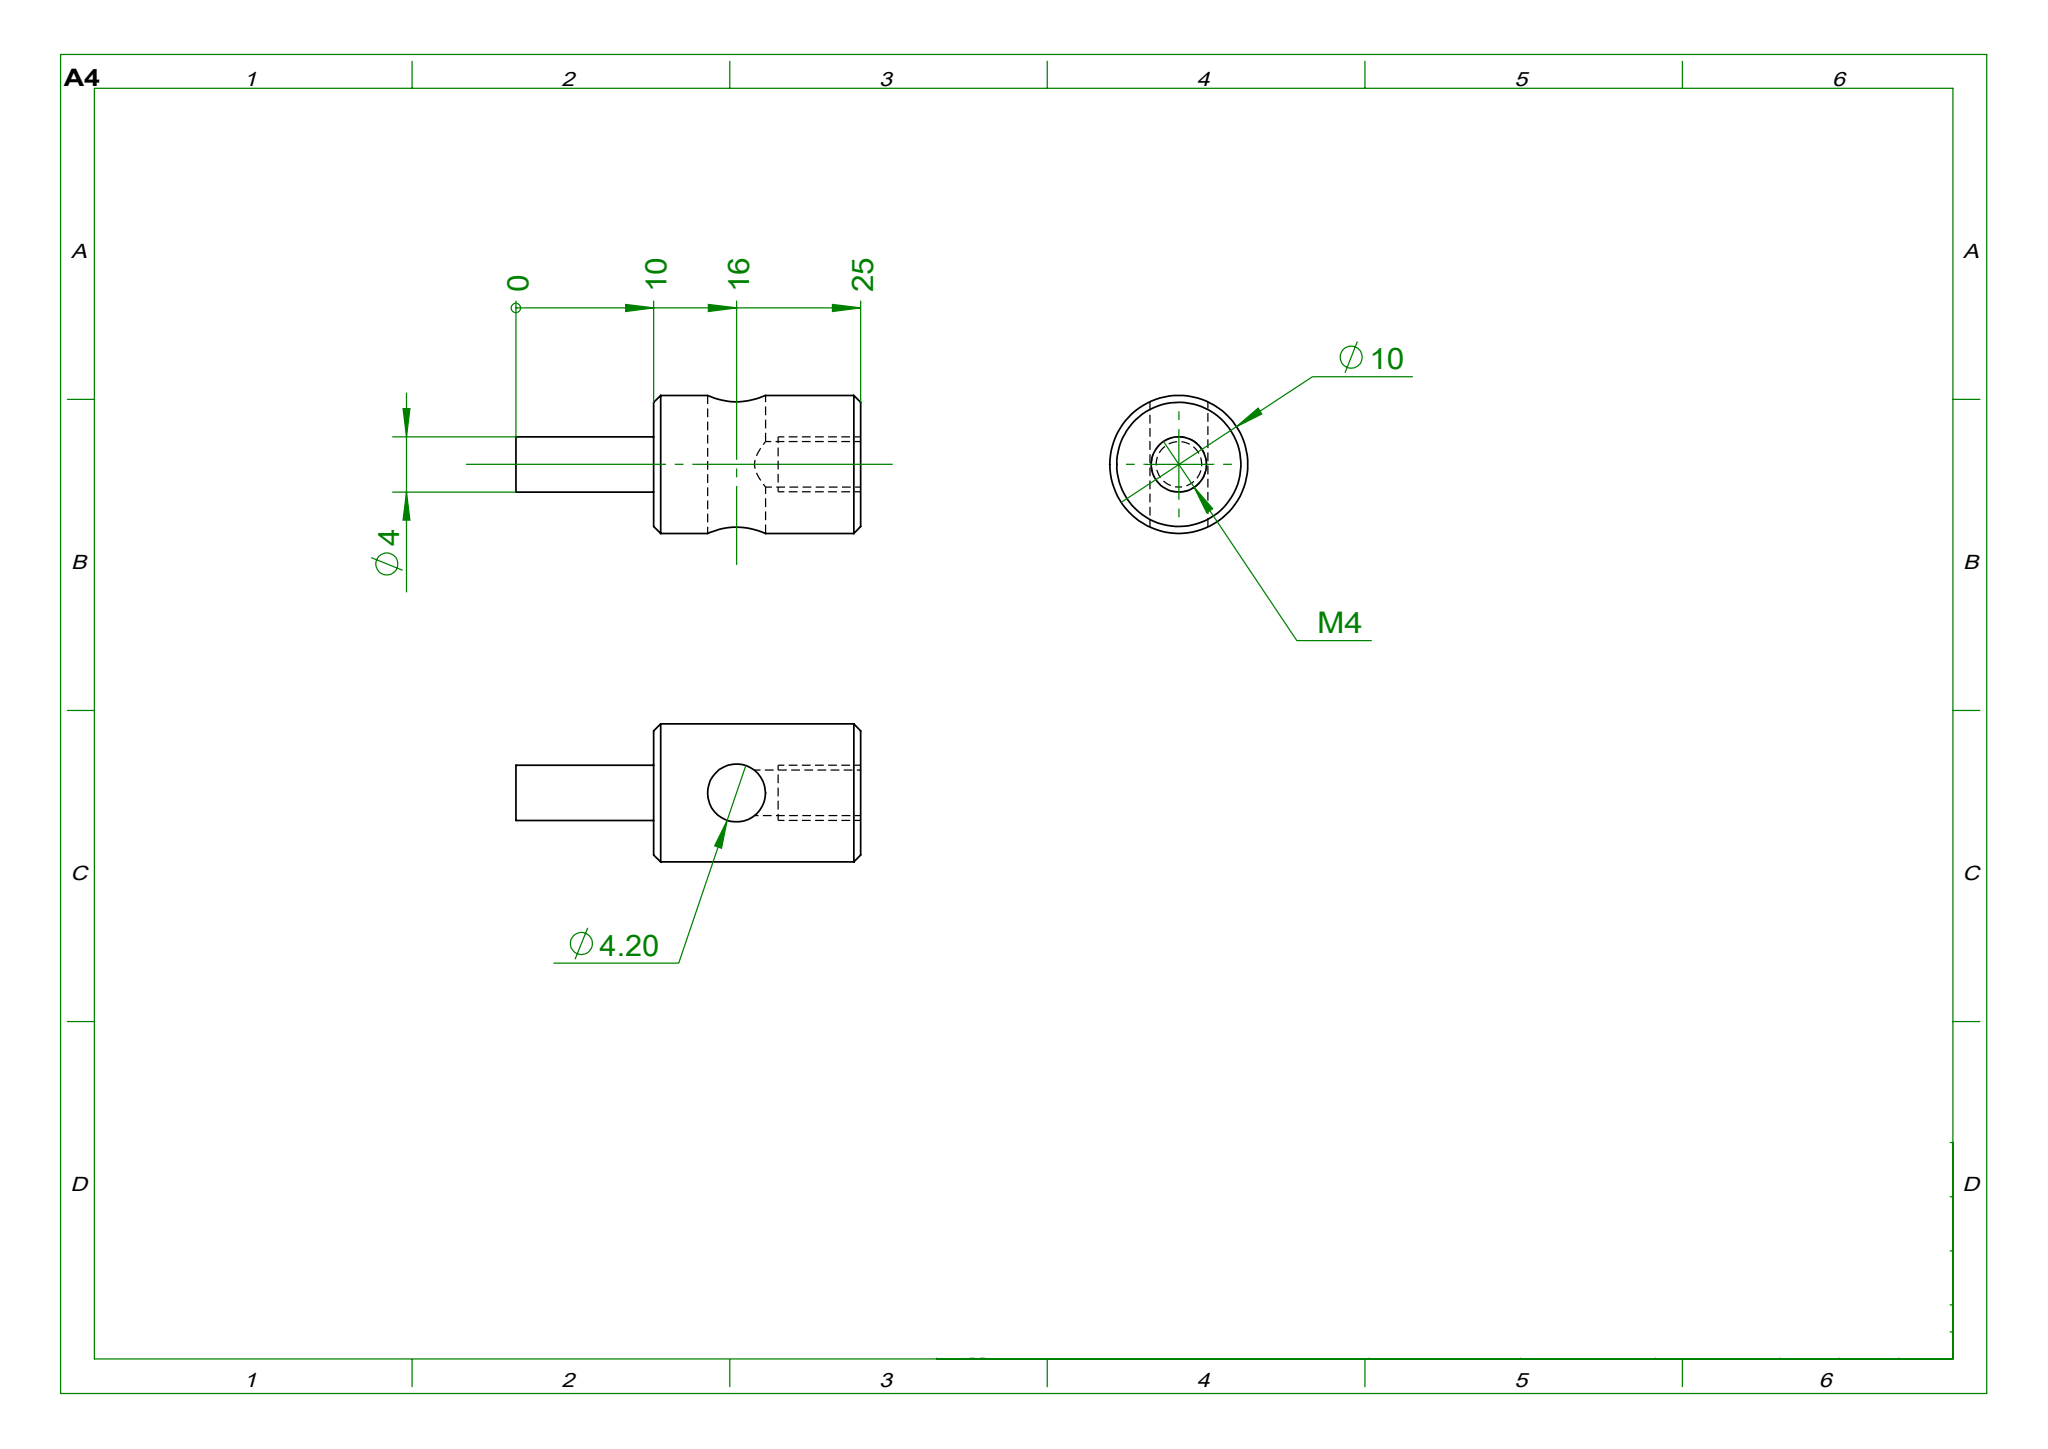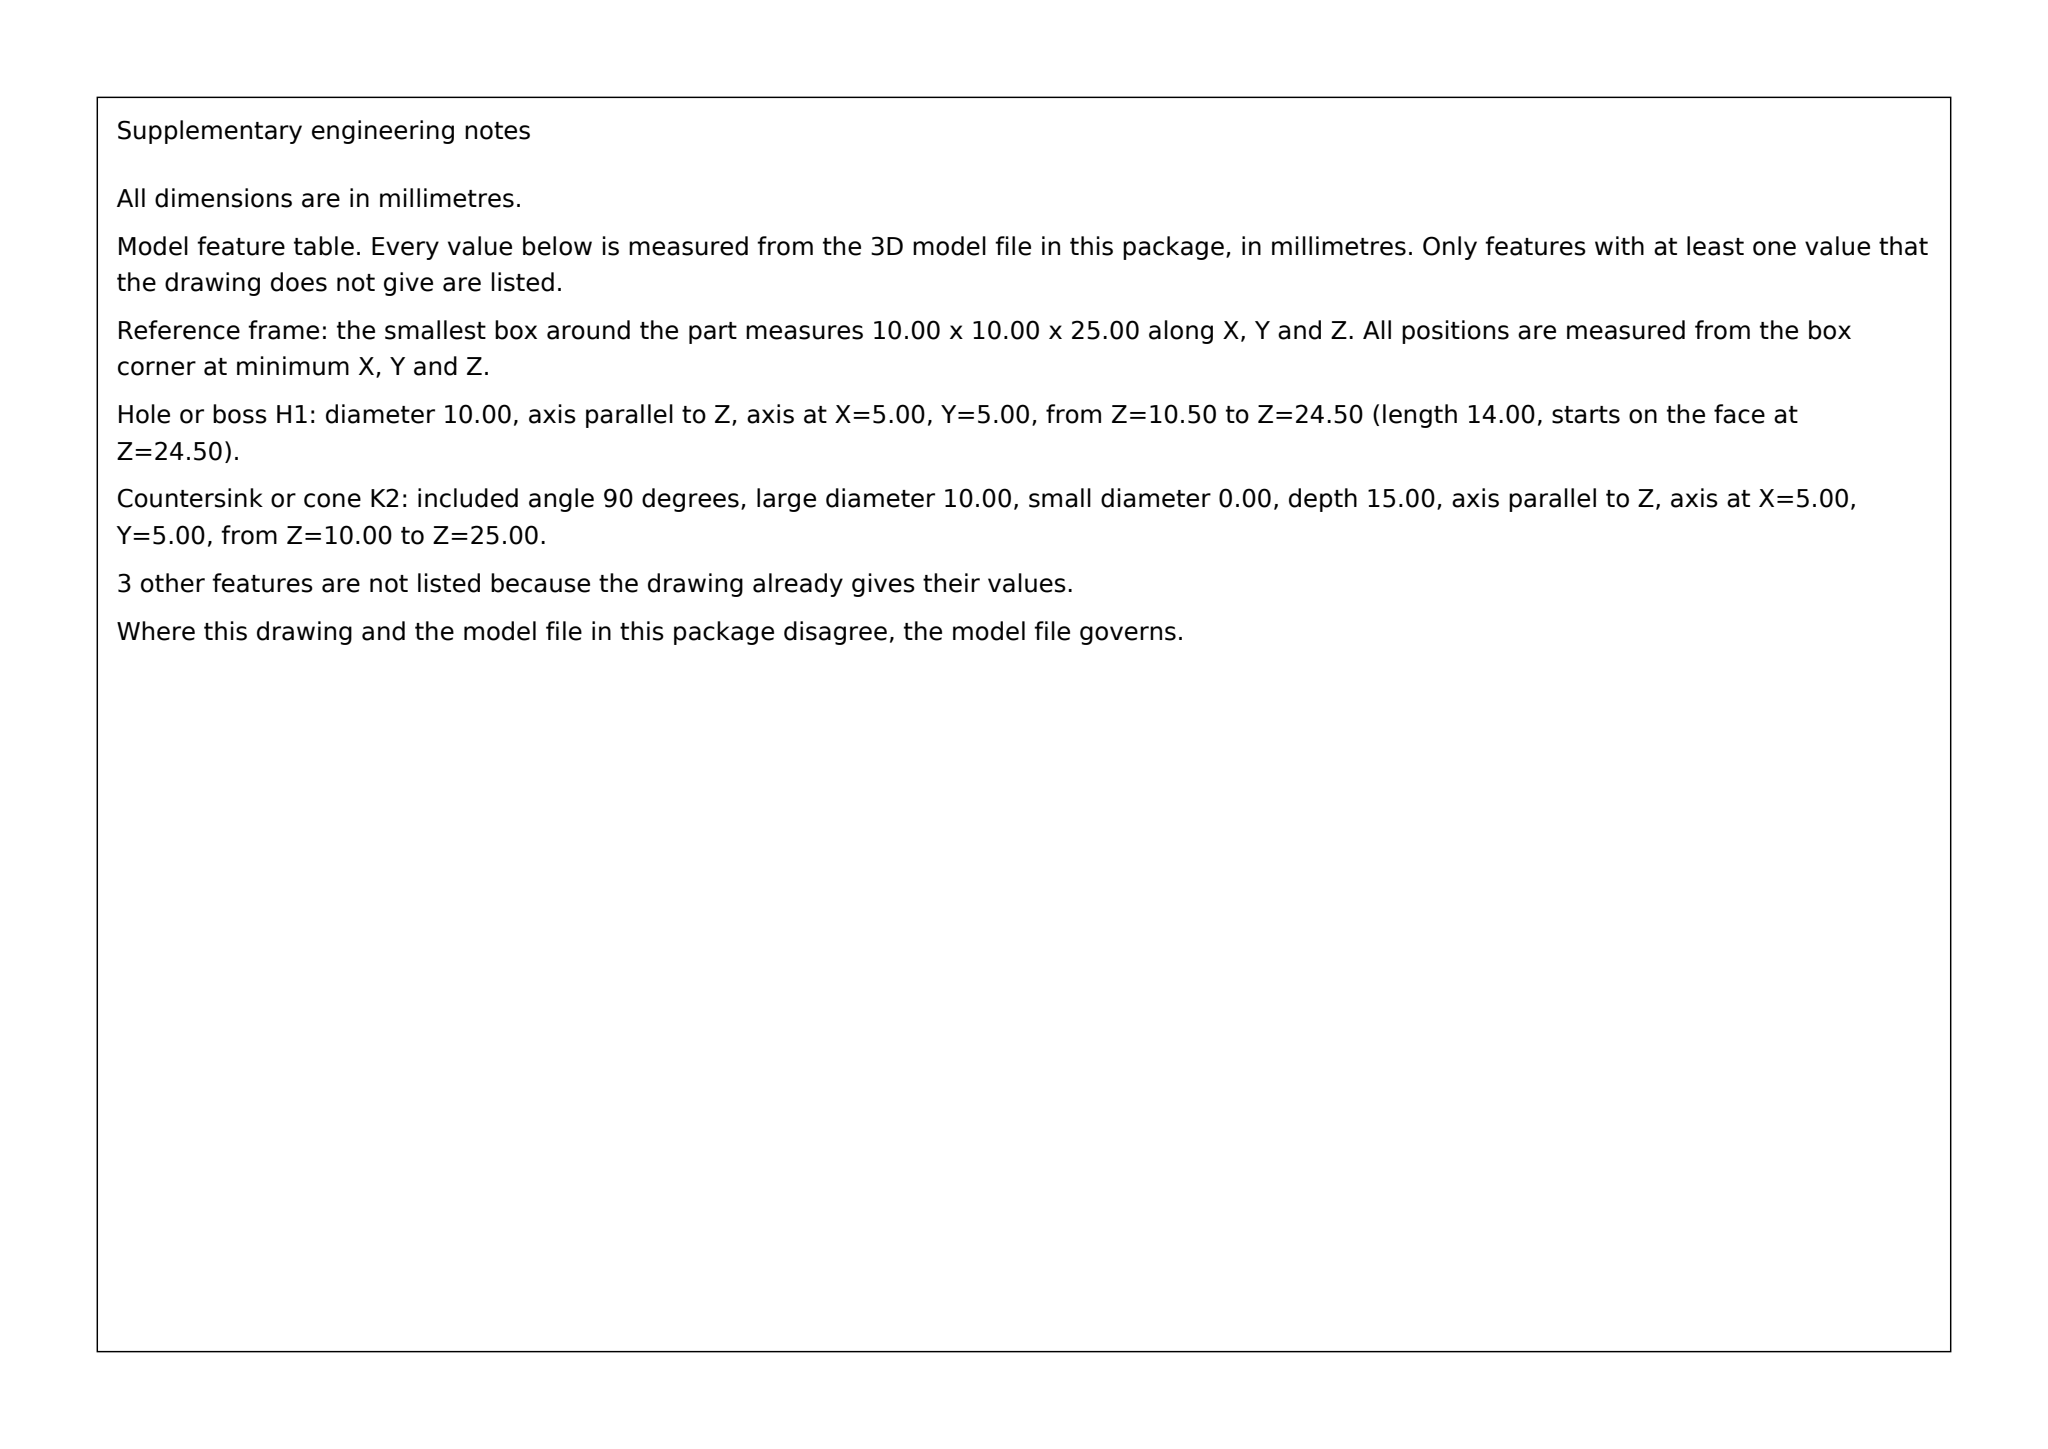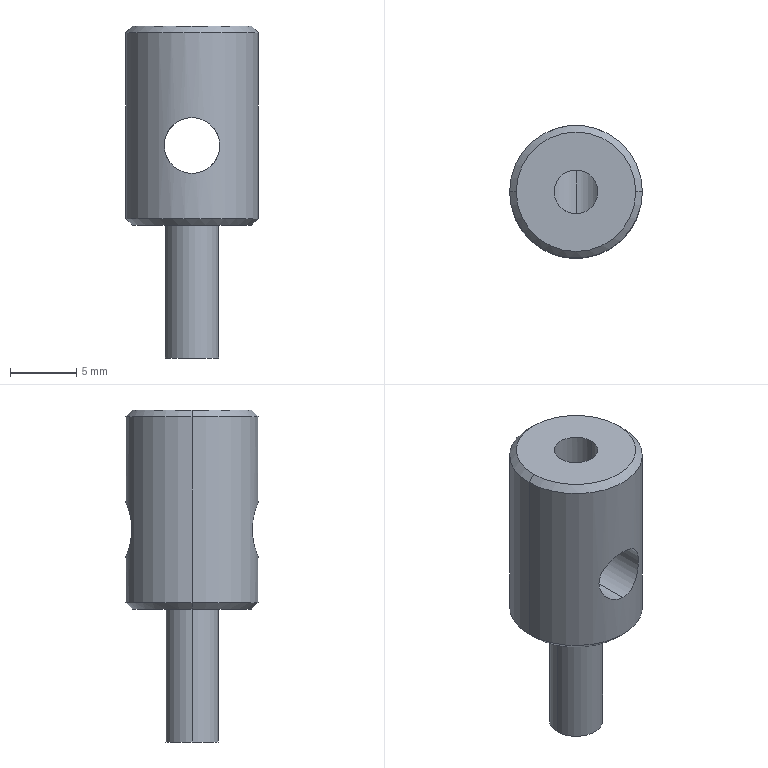Part | SolidWorks | mm | 1 solid | 15 faces | box 10 x 10 x 25 mm | volume 1100 mm3 | cylinder 8 | cone 4 | plane 3 | commonest cylinder face diameters 3.3 x2 4.2 x2 10 x2 4 x2
Drawing notes:
M4 DP 7.7, TAP DRILL Ø3.3 DP 7.7 FROM Ø10 END FACE (25) | from the solid: Ø3.3 z-axis cyl at (5,5), L=7.7 from z=25 face; Ø10 end face plane z=25
Ø10 END: CHAMFER 0.5 X 45° (Ø10 TO Ø9) | from the solid: cones 90° incl, ref Ø10 and Ø9 at Ø10 end; Ø10 cyl L=14 over 15 span
UNSPEC CHAMFERS 0.5 X 45°, BREAK SHARP EDGES | from the solid: only 90° included-angle cones Ø10/Ø9 present; no fillet radii in model
build123d program:
from build123d import *

# Parameters (mm, degrees)
SKETCH1_R             = 2
BOSS_EXTRUDE1_DEPTH   = 10
SKETCH2_R             = 5
BOSS_EXTRUDE2_DEPTH   = 15
SKETCH3_R             = 2.1
CUT_EXTRUDE1_DEPTH    = 6
M4_TAPPED_HOLE1_D     = 3.3
M4_TAPPED_HOLE1_DEPTH = 8
M4_TAPPED_HOLE1_TIP   = 0.9914
CHAMFER1_SIZE         = 0.5


with BuildPart() as part:
    # Sketch1 → Boss-Extrude1 (new body)
    with BuildSketch(Plane.XY):
        Circle(SKETCH1_R)
    extrude(amount=BOSS_EXTRUDE1_DEPTH)

    # Sketch2 → Boss-Extrude2 (add)
    with BuildSketch(Plane.XY.offset(10)):
        Circle(SKETCH2_R)
    extrude(amount=BOSS_EXTRUDE2_DEPTH)

    # Sketch3 → Cut-Extrude1 (cut, symmetric)
    with BuildSketch(Plane(origin=(0, 0, 0), x_dir=(1, 0, 0), z_dir=(0, 1, 0))):
        with Locations(Location((0, -16, 0), (0, 0, 270))):
            Circle(SKETCH3_R)
    extrude(amount=CUT_EXTRUDE1_DEPTH, both=True, mode=Mode.SUBTRACT)

    # M4 Tapped Hole1
    with Locations(Plane.XY.offset(25)):
        with Locations((0, 0)):
            Hole(M4_TAPPED_HOLE1_D / 2, depth=M4_TAPPED_HOLE1_DEPTH)
            with Locations((0, 0, -(M4_TAPPED_HOLE1_DEPTH + M4_TAPPED_HOLE1_TIP / 2))):  # 118° drill point
                Cone(0, M4_TAPPED_HOLE1_D / 2, M4_TAPPED_HOLE1_TIP, mode=Mode.SUBTRACT)

    # Chamfer1
    chamfer1_edges = [part.edges().sort_by_distance(p)[0] for p in [
        (-5, 0, 10),
        (-5, 0, 25),
    ]]
    chamfer(chamfer1_edges, length=CHAMFER1_SIZE)


solid = part.part
STEP:
#1=CARTESIAN_POINT('',(-4.5,0.,10.));
#2=VERTEX_POINT('',#1);
#3=CARTESIAN_POINT('',(4.5,0.,10.));
#4=VERTEX_POINT('',#3);
#5=CARTESIAN_POINT('',(0.,0.,10.));
#6=DIRECTION('',(0.,0.,-1.));
#7=DIRECTION('',(1.,0.,0.));
#8=AXIS2_PLACEMENT_3D('',#5,#6,#7);
#9=CIRCLE('',#8,4.5);
#10=EDGE_CURVE('',#2,#4,#9,.T.);
#11=ORIENTED_EDGE('',*,*,#10,.F.);
#12=CARTESIAN_POINT('',(-5.,0.,10.5));
#13=VERTEX_POINT('',#12);
#14=CARTESIAN_POINT('',(-5.,0.,10.5));
#15=DIRECTION('',(-0.7071,0.,0.7071));
#16=VECTOR('',#15,1000.);
#17=LINE('',#14,#16);
#18=EDGE_CURVE('',#2,#13,#17,.T.);
#19=ORIENTED_EDGE('',*,*,#18,.T.);
#20=CARTESIAN_POINT('',(5.,0.,10.5));
#21=VERTEX_POINT('',#20);
#22=CARTESIAN_POINT('',(0.,0.,10.5));
#23=DIRECTION('',(0.,0.,1.));
#24=DIRECTION('',(1.,0.,0.));
#25=AXIS2_PLACEMENT_3D('',#22,#23,#24);
#26=CIRCLE('',#25,5.);
#27=EDGE_CURVE('',#21,#13,#26,.T.);
#28=ORIENTED_EDGE('',*,*,#27,.F.);
#29=CARTESIAN_POINT('',(5.,0.,10.5));
#30=DIRECTION('',(0.7071,0.,0.7071));
#31=VECTOR('',#30,1000.);
#32=LINE('',#29,#31);
#33=EDGE_CURVE('',#4,#21,#32,.T.);
#34=ORIENTED_EDGE('',*,*,#33,.F.);
#35=EDGE_LOOP('',(#11,#19,#28,#34));
#36=FACE_OUTER_BOUND('',#35,.T.);
#37=CARTESIAN_POINT('',(0.,0.,10.5));
#38=DIRECTION('',(0.,0.,1.));
#39=DIRECTION('',(1.,0.,0.));
#40=AXIS2_PLACEMENT_3D('',#37,#38,#39);
#41=CONICAL_SURFACE('',#40,5.,0.7854);
#42=ADVANCED_FACE('',(#36),#41,.T.);
#43=CARTESIAN_POINT('',(4.5,0.,25.));
#44=VERTEX_POINT('',#43);
#45=CARTESIAN_POINT('',(-4.5,0.,25.));
#46=VERTEX_POINT('',#45);
#47=CARTESIAN_POINT('',(0.,0.,25.));
#48=DIRECTION('',(0.,0.,1.));
#49=DIRECTION('',(1.,0.,0.));
#50=AXIS2_PLACEMENT_3D('',#47,#48,#49);
#51=CIRCLE('',#50,4.5);
#52=EDGE_CURVE('',#44,#46,#51,.T.);
#53=ORIENTED_EDGE('',*,*,#52,.F.);
#54=CARTESIAN_POINT('',(5.,0.,24.5));
#55=VERTEX_POINT('',#54);
#56=CARTESIAN_POINT('',(4.5,0.,25.));
#57=DIRECTION('',(0.7071,0.,-0.7071));
#58=VECTOR('',#57,1000.);
#59=LINE('',#56,#58);
#60=EDGE_CURVE('',#44,#55,#59,.T.);
#61=ORIENTED_EDGE('',*,*,#60,.T.);
#62=CARTESIAN_POINT('',(-5.,0.,24.5));
#63=VERTEX_POINT('',#62);
#64=CARTESIAN_POINT('',(0.,0.,24.5));
#65=DIRECTION('',(0.,0.,-1.));
#66=DIRECTION('',(1.,0.,0.));
#67=AXIS2_PLACEMENT_3D('',#64,#65,#66);
#68=CIRCLE('',#67,5.);
#69=EDGE_CURVE('',#63,#55,#68,.T.);
#70=ORIENTED_EDGE('',*,*,#69,.F.);
#71=CARTESIAN_POINT('',(-4.5,0.,25.));
#72=DIRECTION('',(-0.7071,0.,-0.7071));
#73=VECTOR('',#72,1000.);
#74=LINE('',#71,#73);
#75=EDGE_CURVE('',#46,#63,#74,.T.);
#76=ORIENTED_EDGE('',*,*,#75,.F.);
#77=EDGE_LOOP('',(#53,#61,#70,#76));
#78=FACE_OUTER_BOUND('',#77,.T.);
#79=CARTESIAN_POINT('',(0.,0.,25.));
#80=DIRECTION('',(0.,0.,-1.));
#81=DIRECTION('',(-1.,0.,0.));
#82=AXIS2_PLACEMENT_3D('',#79,#80,#81);
#83=CONICAL_SURFACE('',#82,4.5,0.7854);
#84=ADVANCED_FACE('',(#78),#83,.T.);
#85=CARTESIAN_POINT('',(-1.65,0.,17.299));
#86=VERTEX_POINT('',#85);
#87=CARTESIAN_POINT('',(-0.,-1.65,18.1));
#88=VERTEX_POINT('',#87);
#89=CARTESIAN_POINT('',(-1.65,0.,17.299));
#90=CARTESIAN_POINT('',(-1.65,-0.1142,17.299));
#91=CARTESIAN_POINT('',(-1.638,-0.2279,17.315));
#92=CARTESIAN_POINT('',(-1.592,-0.4459,17.369));
#93=CARTESIAN_POINT('',(-1.56,-0.5481,17.407));
#94=CARTESIAN_POINT('',(-1.436,-0.8406,17.537));
#95=CARTESIAN_POINT('',(-1.321,-1.01,17.642));
#96=CARTESIAN_POINT('',(-1.031,-1.305,17.838));
#97=CARTESIAN_POINT('',(-0.8598,-1.425,17.928));
#98=CARTESIAN_POINT('',(-0.5575,-1.557,18.027));
#99=CARTESIAN_POINT('',(-0.4511,-1.591,18.054));
#100=CARTESIAN_POINT('',(-0.2308,-1.638,18.09));
#101=CARTESIAN_POINT('',(-0.1152,-1.65,18.1));
#102=CARTESIAN_POINT('',(-0.,-1.65,18.1));
#103=B_SPLINE_CURVE_WITH_KNOTS('',3,(#89,#90,#91,#92,#93,#94,#95,#96,#97,#98,#99,#100,#101,#102),.UNSPECIFIED.,.F.,.F.,(4,2,2,2,2,2,4),(0.008161,0.008501,0.00884,0.00952,0.0102,0.01054,0.01088),.UNSPECIFIED.);
#104=EDGE_CURVE('',#86,#88,#103,.T.);
#105=ORIENTED_EDGE('',*,*,#104,.F.);
#106=CARTESIAN_POINT('',(-1.65,0.,25.));
#107=VERTEX_POINT('',#106);
#108=CARTESIAN_POINT('',(-1.65,0.,25.));
#109=DIRECTION('',(0.,0.,1.));
#110=VECTOR('',#109,1000.);
#111=LINE('',#108,#110);
#112=EDGE_CURVE('',#86,#107,#111,.T.);
#113=ORIENTED_EDGE('',*,*,#112,.T.);
#114=CARTESIAN_POINT('',(1.65,0.,25.));
#115=VERTEX_POINT('',#114);
#116=CARTESIAN_POINT('',(0.,0.,25.));
#117=DIRECTION('',(0.,0.,1.));
#118=DIRECTION('',(1.,0.,0.));
#119=AXIS2_PLACEMENT_3D('',#116,#117,#118);
#120=CIRCLE('',#119,1.65);
#121=EDGE_CURVE('',#107,#115,#120,.T.);
#122=ORIENTED_EDGE('',*,*,#121,.T.);
#123=CARTESIAN_POINT('',(1.65,0.,17.299));
#124=VERTEX_POINT('',#123);
#125=CARTESIAN_POINT('',(1.65,0.,25.));
#126=DIRECTION('',(0.,0.,1.));
#127=VECTOR('',#126,1000.);
#128=LINE('',#125,#127);
#129=EDGE_CURVE('',#124,#115,#128,.T.);
#130=ORIENTED_EDGE('',*,*,#129,.F.);
#131=CARTESIAN_POINT('',(-0.,-1.65,18.1));
#132=CARTESIAN_POINT('',(0.1154,-1.65,18.1));
#133=CARTESIAN_POINT('',(0.2279,-1.638,18.091));
#134=CARTESIAN_POINT('',(0.4479,-1.592,18.055));
#135=CARTESIAN_POINT('',(0.5557,-1.557,18.028));
#136=CARTESIAN_POINT('',(0.7557,-1.471,17.962));
#137=CARTESIAN_POINT('',(0.8503,-1.418,17.923));
#138=CARTESIAN_POINT('',(1.024,-1.298,17.836));
#139=CARTESIAN_POINT('',(1.103,-1.231,17.789));
#140=CARTESIAN_POINT('',(1.247,-1.085,17.692));
#141=CARTESIAN_POINT('',(1.313,-1.005,17.641));
#142=CARTESIAN_POINT('',(1.427,-0.8341,17.542));
#143=CARTESIAN_POINT('',(1.477,-0.7439,17.494));
#144=CARTESIAN_POINT('',(1.559,-0.5506,17.408));
#145=CARTESIAN_POINT('',(1.592,-0.4461,17.369));
#146=CARTESIAN_POINT('',(1.638,-0.2292,17.315));
#147=CARTESIAN_POINT('',(1.65,-0.114,17.299));
#148=CARTESIAN_POINT('',(1.65,0.,17.299));
#149=B_SPLINE_CURVE_WITH_KNOTS('',3,(#131,#132,#133,#134,#135,#136,#137,#138,#139,#140,#141,#142,#143,#144,#145,#146,#147,#148),.UNSPECIFIED.,.F.,.F.,(4,2,2,2,2,2,2,2,4),(0.,0.0003404,0.0006807,0.001021,0.001361,0.001702,0.002042,0.002383,0.002723),.UNSPECIFIED.);
#150=EDGE_CURVE('',#88,#124,#149,.T.);
#151=ORIENTED_EDGE('',*,*,#150,.F.);
#152=EDGE_LOOP('',(#105,#113,#122,#130,#151));
#153=FACE_OUTER_BOUND('',#152,.T.);
#154=CARTESIAN_POINT('',(0.,0.,25.));
#155=DIRECTION('',(0.,0.,1.));
#156=DIRECTION('',(1.,0.,0.));
#157=AXIS2_PLACEMENT_3D('',#154,#155,#156);
#158=CYLINDRICAL_SURFACE('',#157,1.65);
#159=ADVANCED_FACE('',(#153),#158,.F.);
#160=CARTESIAN_POINT('',(0.,-5.,13.9));
#161=VERTEX_POINT('',#160);
#162=CARTESIAN_POINT('',(0.,-5.,18.1));
#163=VERTEX_POINT('',#162);
#164=CARTESIAN_POINT('',(0.,-5.,13.9));
#165=CARTESIAN_POINT('',(-0.1383,-5.,13.9));
#166=CARTESIAN_POINT('',(-0.2787,-4.994,13.914));
#167=CARTESIAN_POINT('',(-0.5508,-4.971,13.969));
#168=CARTESIAN_POINT('',(-0.6823,-4.955,14.009));
#169=CARTESIAN_POINT('',(-0.9366,-4.913,14.115));
#170=CARTESIAN_POINT('',(-1.059,-4.888,14.181));
#171=CARTESIAN_POINT('',(-1.284,-4.834,14.333));
#172=CARTESIAN_POINT('',(-1.39,-4.804,14.42));
#173=CARTESIAN_POINT('',(-1.583,-4.744,14.613));
#174=CARTESIAN_POINT('',(-1.668,-4.714,14.718));
#175=CARTESIAN_POINT('',(-1.82,-4.658,14.943));
#176=CARTESIAN_POINT('',(-1.885,-4.631,15.065));
#177=CARTESIAN_POINT('',(-1.991,-4.587,15.318));
#178=CARTESIAN_POINT('',(-2.031,-4.569,15.449));
#179=CARTESIAN_POINT('',(-2.086,-4.544,15.72));
#180=CARTESIAN_POINT('',(-2.1,-4.538,15.861));
#181=CARTESIAN_POINT('',(-2.1,-4.538,16.276));
#182=CARTESIAN_POINT('',(-2.044,-4.565,16.555));
#183=CARTESIAN_POINT('',(-1.886,-4.631,16.935));
#184=CARTESIAN_POINT('',(-1.82,-4.658,17.057));
#185=CARTESIAN_POINT('',(-1.668,-4.714,17.283));
#186=CARTESIAN_POINT('',(-1.582,-4.744,17.388));
#187=CARTESIAN_POINT('',(-1.389,-4.804,17.581));
#188=CARTESIAN_POINT('',(-1.283,-4.834,17.668));
#189=CARTESIAN_POINT('',(-1.058,-4.888,17.819));
#190=CARTESIAN_POINT('',(-0.9378,-4.913,17.884));
#191=CARTESIAN_POINT('',(-0.6819,-4.955,17.991));
#192=CARTESIAN_POINT('',(-0.5504,-4.971,18.031));
#193=CARTESIAN_POINT('',(-0.2803,-4.994,18.086));
#194=CARTESIAN_POINT('',(-0.1404,-5.,18.1));
#195=CARTESIAN_POINT('',(0.,-5.,18.1));
#196=B_SPLINE_CURVE_WITH_KNOTS('',3,(#164,#165,#166,#167,#168,#169,#170,#171,#172,#173,#174,#175,#176,#177,#178,#179,#180,#181,#182,#183,#184,#185,#186,#187,#188,#189,#190,#191,#192,#193,#194,#195),.UNSPECIFIED.,.F.,.F.,(4,2,2,2,2,2,2,2,2,2,2,2,2,2,2,4),(0.006644,0.007058,0.007473,0.007888,0.008303,0.008718,0.009133,0.009548,0.009963,0.01079,0.01121,0.01162,0.01204,0.01245,0.01287,0.01328),.UNSPECIFIED.);
#197=EDGE_CURVE('',#161,#163,#196,.T.);
#198=ORIENTED_EDGE('',*,*,#197,.F.);
#199=CARTESIAN_POINT('',(0.,5.,13.9));
#200=VERTEX_POINT('',#199);
#201=CARTESIAN_POINT('',(0.,-6.,13.9));
#202=DIRECTION('',(0.,1.,0.));
#203=VECTOR('',#202,1000.);
#204=LINE('',#201,#203);
#205=EDGE_CURVE('',#161,#200,#204,.T.);
#206=ORIENTED_EDGE('',*,*,#205,.T.);
#207=CARTESIAN_POINT('',(0.,5.,18.1));
#208=VERTEX_POINT('',#207);
#209=CARTESIAN_POINT('',(0.,5.,18.1));
#210=CARTESIAN_POINT('',(-0.1405,5.,18.1));
#211=CARTESIAN_POINT('',(-0.2784,4.994,18.086));
#212=CARTESIAN_POINT('',(-0.5491,4.972,18.032));
#213=CARTESIAN_POINT('',(-0.6834,4.955,17.99));
#214=CARTESIAN_POINT('',(-0.9371,4.913,17.884));
#215=CARTESIAN_POINT('',(-1.057,4.888,17.82));
#216=CARTESIAN_POINT('',(-1.284,4.834,17.667));
#217=CARTESIAN_POINT('',(-1.39,4.804,17.58));
#218=CARTESIAN_POINT('',(-1.677,4.715,17.292));
#219=CARTESIAN_POINT('',(-1.833,4.653,17.061));
#220=CARTESIAN_POINT('',(-1.99,4.587,16.683));
#221=CARTESIAN_POINT('',(-2.032,4.569,16.549));
#222=CARTESIAN_POINT('',(-2.086,4.544,16.278));
#223=CARTESIAN_POINT('',(-2.1,4.538,16.14));
#224=CARTESIAN_POINT('',(-2.1,4.538,15.863));
#225=CARTESIAN_POINT('',(-2.086,4.544,15.722));
#226=CARTESIAN_POINT('',(-2.032,4.569,15.451));
#227=CARTESIAN_POINT('',(-1.991,4.587,15.319));
#228=CARTESIAN_POINT('',(-1.884,4.632,15.063));
#229=CARTESIAN_POINT('',(-1.82,4.658,14.943));
#230=CARTESIAN_POINT('',(-1.668,4.714,14.717));
#231=CARTESIAN_POINT('',(-1.58,4.745,14.61));
#232=CARTESIAN_POINT('',(-1.388,4.804,14.419));
#233=CARTESIAN_POINT('',(-1.284,4.834,14.333));
#234=CARTESIAN_POINT('',(-1.057,4.888,14.18));
#235=CARTESIAN_POINT('',(-0.9348,4.913,14.115));
#236=CARTESIAN_POINT('',(-0.5563,4.976,13.957));
#237=CARTESIAN_POINT('',(-0.2768,5.,13.9));
#238=CARTESIAN_POINT('',(0.,5.,13.9));
#239=B_SPLINE_CURVE_WITH_KNOTS('',3,(#209,#210,#211,#212,#213,#214,#215,#216,#217,#218,#219,#220,#221,#222,#223,#224,#225,#226,#227,#228,#229,#230,#231,#232,#233,#234,#235,#236,#237,#238),.UNSPECIFIED.,.F.,.F.,(4,2,2,2,2,2,2,2,2,2,2,2,2,2,4),(0.,0.0004152,0.0008304,0.001246,0.001661,0.002491,0.002907,0.003322,0.003737,0.004152,0.004567,0.004983,0.005398,0.005813,0.006644),.UNSPECIFIED.);
#240=EDGE_CURVE('',#208,#200,#239,.T.);
#241=ORIENTED_EDGE('',*,*,#240,.F.);
#242=CARTESIAN_POINT('',(0.,1.65,18.1));
#243=VERTEX_POINT('',#242);
#244=CARTESIAN_POINT('',(0.,-6.,18.1));
#245=DIRECTION('',(0.,1.,0.));
#246=VECTOR('',#245,1000.);
#247=LINE('',#244,#246);
#248=EDGE_CURVE('',#243,#208,#247,.T.);
#249=ORIENTED_EDGE('',*,*,#248,.F.);
#250=CARTESIAN_POINT('',(0.,1.65,18.1));
#251=CARTESIAN_POINT('',(-0.1133,1.65,18.1));
#252=CARTESIAN_POINT('',(-0.2281,1.638,18.091));
#253=CARTESIAN_POINT('',(-0.4485,1.592,18.055));
#254=CARTESIAN_POINT('',(-0.5541,1.558,18.028));
#255=CARTESIAN_POINT('',(-0.8571,1.427,17.929));
#256=CARTESIAN_POINT('',(-1.031,1.304,17.838));
#257=CARTESIAN_POINT('',(-1.32,1.011,17.643));
#258=CARTESIAN_POINT('',(-1.436,0.8397,17.537));
#259=CARTESIAN_POINT('',(-1.559,0.5497,17.408));
#260=CARTESIAN_POINT('',(-1.593,0.4454,17.369));
#261=CARTESIAN_POINT('',(-1.638,0.2287,17.315));
#262=CARTESIAN_POINT('',(-1.65,0.114,17.299));
#263=CARTESIAN_POINT('',(-1.65,0.,17.299));
#264=B_SPLINE_CURVE_WITH_KNOTS('',3,(#250,#251,#252,#253,#254,#255,#256,#257,#258,#259,#260,#261,#262,#263),.UNSPECIFIED.,.F.,.F.,(4,2,2,2,2,2,4),(0.005446,0.005786,0.006125,0.006804,0.007482,0.007822,0.008161),.UNSPECIFIED.);
#265=EDGE_CURVE('',#243,#86,#264,.T.);
#266=ORIENTED_EDGE('',*,*,#265,.T.);
#267=ORIENTED_EDGE('',*,*,#104,.T.);
#268=CARTESIAN_POINT('',(0.,-6.,18.1));
#269=DIRECTION('',(0.,1.,0.));
#270=VECTOR('',#269,1000.);
#271=LINE('',#268,#270);
#272=EDGE_CURVE('',#163,#88,#271,.T.);
#273=ORIENTED_EDGE('',*,*,#272,.F.);
#274=EDGE_LOOP('',(#198,#206,#241,#249,#266,#267,#273));
#275=FACE_OUTER_BOUND('',#274,.T.);
#276=CARTESIAN_POINT('',(0.,-6.,16.));
#277=DIRECTION('',(0.,1.,0.));
#278=DIRECTION('',(0.,0.,1.));
#279=AXIS2_PLACEMENT_3D('',#276,#277,#278);
#280=CYLINDRICAL_SURFACE('',#279,2.1);
#281=ADVANCED_FACE('',(#275),#280,.F.);
#282=ORIENTED_EDGE('',*,*,#240,.T.);
#283=CARTESIAN_POINT('',(0.,5.,13.9));
#284=CARTESIAN_POINT('',(0.1383,5.,13.9));
#285=CARTESIAN_POINT('',(0.2787,4.994,13.914));
#286=CARTESIAN_POINT('',(0.5508,4.971,13.969));
#287=CARTESIAN_POINT('',(0.6823,4.955,14.009));
#288=CARTESIAN_POINT('',(0.9366,4.913,14.115));
#289=CARTESIAN_POINT('',(1.059,4.888,14.181));
#290=CARTESIAN_POINT('',(1.284,4.834,14.333));
#291=CARTESIAN_POINT('',(1.39,4.804,14.42));
#292=CARTESIAN_POINT('',(1.583,4.744,14.613));
#293=CARTESIAN_POINT('',(1.668,4.714,14.718));
#294=CARTESIAN_POINT('',(1.82,4.658,14.943));
#295=CARTESIAN_POINT('',(1.885,4.631,15.065));
#296=CARTESIAN_POINT('',(1.991,4.587,15.318));
#297=CARTESIAN_POINT('',(2.031,4.569,15.449));
#298=CARTESIAN_POINT('',(2.086,4.544,15.72));
#299=CARTESIAN_POINT('',(2.1,4.538,15.861));
#300=CARTESIAN_POINT('',(2.1,4.538,16.276));
#301=CARTESIAN_POINT('',(2.044,4.565,16.555));
#302=CARTESIAN_POINT('',(1.886,4.631,16.935));
#303=CARTESIAN_POINT('',(1.82,4.658,17.057));
#304=CARTESIAN_POINT('',(1.668,4.714,17.283));
#305=CARTESIAN_POINT('',(1.582,4.744,17.388));
#306=CARTESIAN_POINT('',(1.389,4.804,17.581));
#307=CARTESIAN_POINT('',(1.283,4.834,17.668));
#308=CARTESIAN_POINT('',(1.058,4.888,17.819));
#309=CARTESIAN_POINT('',(0.9378,4.913,17.884));
#310=CARTESIAN_POINT('',(0.6819,4.955,17.991));
#311=CARTESIAN_POINT('',(0.5504,4.971,18.031));
#312=CARTESIAN_POINT('',(0.2803,4.994,18.086));
#313=CARTESIAN_POINT('',(0.1404,5.,18.1));
#314=CARTESIAN_POINT('',(0.,5.,18.1));
#315=B_SPLINE_CURVE_WITH_KNOTS('',3,(#283,#284,#285,#286,#287,#288,#289,#290,#291,#292,#293,#294,#295,#296,#297,#298,#299,#300,#301,#302,#303,#304,#305,#306,#307,#308,#309,#310,#311,#312,#313,#314),.UNSPECIFIED.,.F.,.F.,(4,2,2,2,2,2,2,2,2,2,2,2,2,2,2,4),(0.006644,0.007058,0.007473,0.007888,0.008303,0.008718,0.009133,0.009548,0.009963,0.01079,0.01121,0.01162,0.01204,0.01245,0.01287,0.01328),.UNSPECIFIED.);
#316=EDGE_CURVE('',#200,#208,#315,.T.);
#317=ORIENTED_EDGE('',*,*,#316,.T.);
#318=EDGE_LOOP('',(#282,#317));
#319=FACE_BOUND('',#318,.T.);
#320=ORIENTED_EDGE('',*,*,#69,.T.);
#321=CARTESIAN_POINT('',(5.,0.,25.));
#322=DIRECTION('',(0.,0.,-1.));
#323=VECTOR('',#322,1000.);
#324=LINE('',#321,#323);
#325=EDGE_CURVE('',#55,#21,#324,.T.);
#326=ORIENTED_EDGE('',*,*,#325,.T.);
#327=ORIENTED_EDGE('',*,*,#27,.T.);
#328=CARTESIAN_POINT('',(-5.,0.,25.));
#329=DIRECTION('',(0.,0.,-1.));
#330=VECTOR('',#329,1000.);
#331=LINE('',#328,#330);
#332=EDGE_CURVE('',#63,#13,#331,.T.);
#333=ORIENTED_EDGE('',*,*,#332,.F.);
#334=EDGE_LOOP('',(#320,#326,#327,#333));
#335=FACE_OUTER_BOUND('',#334,.T.);
#336=CARTESIAN_POINT('',(0.,0.,25.));
#337=DIRECTION('',(0.,0.,-1.));
#338=DIRECTION('',(-1.,0.,0.));
#339=AXIS2_PLACEMENT_3D('',#336,#337,#338);
#340=CYLINDRICAL_SURFACE('',#339,5.);
#341=ADVANCED_FACE('',(#319,#335),#340,.T.);
#342=CARTESIAN_POINT('',(2.,0.,10.));
#343=VERTEX_POINT('',#342);
#344=CARTESIAN_POINT('',(-2.,0.,10.));
#345=VERTEX_POINT('',#344);
#346=CARTESIAN_POINT('',(0.,0.,10.));
#347=DIRECTION('',(0.,0.,1.));
#348=DIRECTION('',(1.,0.,0.));
#349=AXIS2_PLACEMENT_3D('',#346,#347,#348);
#350=CIRCLE('',#349,2.);
#351=EDGE_CURVE('',#343,#345,#350,.T.);
#352=ORIENTED_EDGE('',*,*,#351,.F.);
#353=CARTESIAN_POINT('',(2.,0.,0.));
#354=VERTEX_POINT('',#353);
#355=CARTESIAN_POINT('',(2.,0.,10.));
#356=DIRECTION('',(0.,0.,-1.));
#357=VECTOR('',#356,1000.);
#358=LINE('',#355,#357);
#359=EDGE_CURVE('',#343,#354,#358,.T.);
#360=ORIENTED_EDGE('',*,*,#359,.T.);
#361=CARTESIAN_POINT('',(-2.,0.,0.));
#362=VERTEX_POINT('',#361);
#363=CARTESIAN_POINT('',(0.,0.,0.));
#364=DIRECTION('',(0.,0.,1.));
#365=DIRECTION('',(1.,0.,0.));
#366=AXIS2_PLACEMENT_3D('',#363,#364,#365);
#367=CIRCLE('',#366,2.);
#368=EDGE_CURVE('',#354,#362,#367,.T.);
#369=ORIENTED_EDGE('',*,*,#368,.T.);
#370=CARTESIAN_POINT('',(-2.,0.,10.));
#371=DIRECTION('',(0.,0.,-1.));
#372=VECTOR('',#371,1000.);
#373=LINE('',#370,#372);
#374=EDGE_CURVE('',#345,#362,#373,.T.);
#375=ORIENTED_EDGE('',*,*,#374,.F.);
#376=EDGE_LOOP('',(#352,#360,#369,#375));
#377=FACE_OUTER_BOUND('',#376,.T.);
#378=CARTESIAN_POINT('',(0.,0.,10.));
#379=DIRECTION('',(0.,0.,-1.));
#380=DIRECTION('',(-1.,0.,0.));
#381=AXIS2_PLACEMENT_3D('',#378,#379,#380);
#382=CYLINDRICAL_SURFACE('',#381,2.);
#383=ADVANCED_FACE('',(#377),#382,.T.);
#384=ORIENTED_EDGE('',*,*,#359,.F.);
#385=CARTESIAN_POINT('',(0.,0.,10.));
#386=DIRECTION('',(0.,0.,1.));
#387=DIRECTION('',(1.,0.,0.));
#388=AXIS2_PLACEMENT_3D('',#385,#386,#387);
#389=CIRCLE('',#388,2.);
#390=EDGE_CURVE('',#345,#343,#389,.T.);
#391=ORIENTED_EDGE('',*,*,#390,.F.);
#392=ORIENTED_EDGE('',*,*,#374,.T.);
#393=CARTESIAN_POINT('',(0.,0.,0.));
#394=DIRECTION('',(0.,0.,1.));
#395=DIRECTION('',(1.,0.,0.));
#396=AXIS2_PLACEMENT_3D('',#393,#394,#395);
#397=CIRCLE('',#396,2.);
#398=EDGE_CURVE('',#362,#354,#397,.T.);
#399=ORIENTED_EDGE('',*,*,#398,.T.);
#400=EDGE_LOOP('',(#384,#391,#392,#399));
#401=FACE_OUTER_BOUND('',#400,.T.);
#402=CARTESIAN_POINT('',(0.,0.,10.));
#403=DIRECTION('',(0.,0.,-1.));
#404=DIRECTION('',(-1.,0.,0.));
#405=AXIS2_PLACEMENT_3D('',#402,#403,#404);
#406=CYLINDRICAL_SURFACE('',#405,2.);
#407=ADVANCED_FACE('',(#401),#406,.T.);
#408=ORIENTED_EDGE('',*,*,#398,.F.);
#409=ORIENTED_EDGE('',*,*,#368,.F.);
#410=EDGE_LOOP('',(#408,#409));
#411=FACE_OUTER_BOUND('',#410,.T.);
#412=CARTESIAN_POINT('',(0.,0.,0.));
#413=DIRECTION('',(0.,0.,1.));
#414=DIRECTION('',(1.,0.,0.));
#415=AXIS2_PLACEMENT_3D('',#412,#413,#414);
#416=PLANE('',#415);
#417=ADVANCED_FACE('',(#411),#416,.F.);
#418=CARTESIAN_POINT('',(0.,0.,10.));
#419=DIRECTION('',(0.,0.,-1.));
#420=DIRECTION('',(1.,0.,0.));
#421=AXIS2_PLACEMENT_3D('',#418,#419,#420);
#422=CIRCLE('',#421,4.5);
#423=EDGE_CURVE('',#4,#2,#422,.T.);
#424=ORIENTED_EDGE('',*,*,#423,.T.);
#425=ORIENTED_EDGE('',*,*,#10,.T.);
#426=EDGE_LOOP('',(#424,#425));
#427=FACE_OUTER_BOUND('',#426,.T.);
#428=ORIENTED_EDGE('',*,*,#390,.T.);
#429=ORIENTED_EDGE('',*,*,#351,.T.);
#430=EDGE_LOOP('',(#428,#429));
#431=FACE_BOUND('',#430,.T.);
#432=CARTESIAN_POINT('',(0.,0.,10.));
#433=DIRECTION('',(0.,0.,1.));
#434=DIRECTION('',(1.,0.,0.));
#435=AXIS2_PLACEMENT_3D('',#432,#433,#434);
#436=PLANE('',#435);
#437=ADVANCED_FACE('',(#427,#431),#436,.F.);
#438=ORIENTED_EDGE('',*,*,#325,.F.);
#439=CARTESIAN_POINT('',(0.,0.,24.5));
#440=DIRECTION('',(0.,0.,-1.));
#441=DIRECTION('',(1.,0.,0.));
#442=AXIS2_PLACEMENT_3D('',#439,#440,#441);
#443=CIRCLE('',#442,5.);
#444=EDGE_CURVE('',#55,#63,#443,.T.);
#445=ORIENTED_EDGE('',*,*,#444,.T.);
#446=ORIENTED_EDGE('',*,*,#332,.T.);
#447=CARTESIAN_POINT('',(0.,0.,10.5));
#448=DIRECTION('',(0.,0.,1.));
#449=DIRECTION('',(1.,0.,0.));
#450=AXIS2_PLACEMENT_3D('',#447,#448,#449);
#451=CIRCLE('',#450,5.);
#452=EDGE_CURVE('',#13,#21,#451,.T.);
#453=ORIENTED_EDGE('',*,*,#452,.T.);
#454=EDGE_LOOP('',(#438,#445,#446,#453));
#455=FACE_OUTER_BOUND('',#454,.T.);
#456=CARTESIAN_POINT('',(0.,-5.,18.1));
#457=CARTESIAN_POINT('',(0.1405,-5.,18.1));
#458=CARTESIAN_POINT('',(0.2784,-4.994,18.086));
#459=CARTESIAN_POINT('',(0.5491,-4.972,18.032));
#460=CARTESIAN_POINT('',(0.6834,-4.955,17.99));
#461=CARTESIAN_POINT('',(0.9371,-4.913,17.884));
#462=CARTESIAN_POINT('',(1.057,-4.888,17.82));
#463=CARTESIAN_POINT('',(1.284,-4.834,17.667));
#464=CARTESIAN_POINT('',(1.39,-4.804,17.58));
#465=CARTESIAN_POINT('',(1.677,-4.715,17.292));
#466=CARTESIAN_POINT('',(1.833,-4.653,17.061));
#467=CARTESIAN_POINT('',(1.99,-4.587,16.683));
#468=CARTESIAN_POINT('',(2.032,-4.569,16.549));
#469=CARTESIAN_POINT('',(2.086,-4.544,16.278));
#470=CARTESIAN_POINT('',(2.1,-4.538,16.14));
#471=CARTESIAN_POINT('',(2.1,-4.538,15.863));
#472=CARTESIAN_POINT('',(2.086,-4.544,15.722));
#473=CARTESIAN_POINT('',(2.032,-4.569,15.451));
#474=CARTESIAN_POINT('',(1.991,-4.587,15.319));
#475=CARTESIAN_POINT('',(1.884,-4.632,15.063));
#476=CARTESIAN_POINT('',(1.82,-4.658,14.943));
#477=CARTESIAN_POINT('',(1.668,-4.714,14.717));
#478=CARTESIAN_POINT('',(1.58,-4.745,14.61));
#479=CARTESIAN_POINT('',(1.388,-4.804,14.419));
#480=CARTESIAN_POINT('',(1.284,-4.834,14.333));
#481=CARTESIAN_POINT('',(1.057,-4.888,14.18));
#482=CARTESIAN_POINT('',(0.9348,-4.913,14.115));
#483=CARTESIAN_POINT('',(0.5563,-4.976,13.957));
#484=CARTESIAN_POINT('',(0.2768,-5.,13.9));
#485=CARTESIAN_POINT('',(0.,-5.,13.9));
#486=B_SPLINE_CURVE_WITH_KNOTS('',3,(#456,#457,#458,#459,#460,#461,#462,#463,#464,#465,#466,#467,#468,#469,#470,#471,#472,#473,#474,#475,#476,#477,#478,#479,#480,#481,#482,#483,#484,#485),.UNSPECIFIED.,.F.,.F.,(4,2,2,2,2,2,2,2,2,2,2,2,2,2,4),(0.,0.0004152,0.0008304,0.001246,0.001661,0.002491,0.002907,0.003322,0.003737,0.004152,0.004567,0.004983,0.005398,0.005813,0.006644),.UNSPECIFIED.);
#487=EDGE_CURVE('',#163,#161,#486,.T.);
#488=ORIENTED_EDGE('',*,*,#487,.T.);
#489=ORIENTED_EDGE('',*,*,#197,.T.);
#490=EDGE_LOOP('',(#488,#489));
#491=FACE_BOUND('',#490,.T.);
#492=CARTESIAN_POINT('',(0.,0.,25.));
#493=DIRECTION('',(0.,0.,-1.));
#494=DIRECTION('',(-1.,0.,0.));
#495=AXIS2_PLACEMENT_3D('',#492,#493,#494);
#496=CYLINDRICAL_SURFACE('',#495,5.);
#497=ADVANCED_FACE('',(#455,#491),#496,.T.);
#498=CARTESIAN_POINT('',(0.,0.,25.));
#499=DIRECTION('',(0.,0.,1.));
#500=DIRECTION('',(1.,0.,0.));
#501=AXIS2_PLACEMENT_3D('',#498,#499,#500);
#502=CIRCLE('',#501,4.5);
#503=EDGE_CURVE('',#46,#44,#502,.T.);
#504=ORIENTED_EDGE('',*,*,#503,.T.);
#505=ORIENTED_EDGE('',*,*,#52,.T.);
#506=EDGE_LOOP('',(#504,#505));
#507=FACE_OUTER_BOUND('',#506,.T.);
#508=CARTESIAN_POINT('',(0.,0.,25.));
#509=DIRECTION('',(0.,0.,1.));
#510=DIRECTION('',(1.,0.,0.));
#511=AXIS2_PLACEMENT_3D('',#508,#509,#510);
#512=CIRCLE('',#511,1.65);
#513=EDGE_CURVE('',#115,#107,#512,.T.);
#514=ORIENTED_EDGE('',*,*,#513,.F.);
#515=ORIENTED_EDGE('',*,*,#121,.F.);
#516=EDGE_LOOP('',(#514,#515));
#517=FACE_BOUND('',#516,.T.);
#518=CARTESIAN_POINT('',(0.,0.,25.));
#519=DIRECTION('',(0.,0.,1.));
#520=DIRECTION('',(1.,0.,0.));
#521=AXIS2_PLACEMENT_3D('',#518,#519,#520);
#522=PLANE('',#521);
#523=ADVANCED_FACE('',(#507,#517),#522,.T.);
#524=ORIENTED_EDGE('',*,*,#205,.F.);
#525=ORIENTED_EDGE('',*,*,#487,.F.);
#526=ORIENTED_EDGE('',*,*,#272,.T.);
#527=ORIENTED_EDGE('',*,*,#150,.T.);
#528=CARTESIAN_POINT('',(1.65,0.,17.299));
#529=CARTESIAN_POINT('',(1.65,0.114,17.299));
#530=CARTESIAN_POINT('',(1.638,0.2283,17.315));
#531=CARTESIAN_POINT('',(1.592,0.4459,17.369));
#532=CARTESIAN_POINT('',(1.56,0.5483,17.407));
#533=CARTESIAN_POINT('',(1.435,0.8417,17.538));
#534=CARTESIAN_POINT('',(1.321,1.01,17.642));
#535=CARTESIAN_POINT('',(1.03,1.306,17.839));
#536=CARTESIAN_POINT('',(0.8587,1.426,17.928));
#537=CARTESIAN_POINT('',(0.5554,1.558,18.028));
#538=CARTESIAN_POINT('',(0.4498,1.592,18.054));
#539=CARTESIAN_POINT('',(0.229,1.638,18.09));
#540=CARTESIAN_POINT('',(0.1136,1.65,18.1));
#541=CARTESIAN_POINT('',(0.,1.65,18.1));
#542=B_SPLINE_CURVE_WITH_KNOTS('',3,(#528,#529,#530,#531,#532,#533,#534,#535,#536,#537,#538,#539,#540,#541),.UNSPECIFIED.,.F.,.F.,(4,2,2,2,2,2,4),(0.002723,0.003063,0.003404,0.004085,0.004766,0.005106,0.005446),.UNSPECIFIED.);
#543=EDGE_CURVE('',#124,#243,#542,.T.);
#544=ORIENTED_EDGE('',*,*,#543,.T.);
#545=ORIENTED_EDGE('',*,*,#248,.T.);
#546=ORIENTED_EDGE('',*,*,#316,.F.);
#547=EDGE_LOOP('',(#524,#525,#526,#527,#544,#545,#546));
#548=FACE_OUTER_BOUND('',#547,.T.);
#549=CARTESIAN_POINT('',(0.,-6.,16.));
#550=DIRECTION('',(0.,1.,0.));
#551=DIRECTION('',(0.,0.,1.));
#552=AXIS2_PLACEMENT_3D('',#549,#550,#551);
#553=CYLINDRICAL_SURFACE('',#552,2.1);
#554=ADVANCED_FACE('',(#548),#553,.F.);
#555=ORIENTED_EDGE('',*,*,#112,.F.);
#556=ORIENTED_EDGE('',*,*,#265,.F.);
#557=ORIENTED_EDGE('',*,*,#543,.F.);
#558=ORIENTED_EDGE('',*,*,#129,.T.);
#559=ORIENTED_EDGE('',*,*,#513,.T.);
#560=EDGE_LOOP('',(#555,#556,#557,#558,#559));
#561=FACE_OUTER_BOUND('',#560,.T.);
#562=CARTESIAN_POINT('',(0.,0.,25.));
#563=DIRECTION('',(0.,0.,1.));
#564=DIRECTION('',(1.,0.,0.));
#565=AXIS2_PLACEMENT_3D('',#562,#563,#564);
#566=CYLINDRICAL_SURFACE('',#565,1.65);
#567=ADVANCED_FACE('',(#561),#566,.F.);
#568=ORIENTED_EDGE('',*,*,#60,.F.);
#569=ORIENTED_EDGE('',*,*,#503,.F.);
#570=ORIENTED_EDGE('',*,*,#75,.T.);
#571=ORIENTED_EDGE('',*,*,#444,.F.);
#572=EDGE_LOOP('',(#568,#569,#570,#571));
#573=FACE_OUTER_BOUND('',#572,.T.);
#574=CARTESIAN_POINT('',(0.,0.,25.));
#575=DIRECTION('',(0.,0.,-1.));
#576=DIRECTION('',(-1.,0.,0.));
#577=AXIS2_PLACEMENT_3D('',#574,#575,#576);
#578=CONICAL_SURFACE('',#577,4.5,0.7854);
#579=ADVANCED_FACE('',(#573),#578,.T.);
#580=ORIENTED_EDGE('',*,*,#18,.F.);
#581=ORIENTED_EDGE('',*,*,#423,.F.);
#582=ORIENTED_EDGE('',*,*,#33,.T.);
#583=ORIENTED_EDGE('',*,*,#452,.F.);
#584=EDGE_LOOP('',(#580,#581,#582,#583));
#585=FACE_OUTER_BOUND('',#584,.T.);
#586=CARTESIAN_POINT('',(0.,0.,10.5));
#587=DIRECTION('',(0.,0.,1.));
#588=DIRECTION('',(1.,0.,0.));
#589=AXIS2_PLACEMENT_3D('',#586,#587,#588);
#590=CONICAL_SURFACE('',#589,5.,0.7854);
#591=ADVANCED_FACE('',(#585),#590,.T.);
#592=CLOSED_SHELL('',(#42,#84,#159,#281,#341,#383,#407,#417,#437,#497,#523,#554,#567,#579,#591));
#593=MANIFOLD_SOLID_BREP('',#592);
#594=CARTESIAN_POINT('',(0.,0.,0.));
#595=DIRECTION('',(0.,0.,1.));
#596=DIRECTION('',(1.,0.,0.));
#597=AXIS2_PLACEMENT_3D('',#594,#595,#596);
#598=(LENGTH_UNIT()NAMED_UNIT(*)SI_UNIT(.MILLI.,.METRE.));
#599=UNCERTAINTY_MEASURE_WITH_UNIT(LENGTH_MEASURE(0.00001),#598,'','');
#600=(NAMED_UNIT(*)PLANE_ANGLE_UNIT()SI_UNIT($,.RADIAN.));
#601=(NAMED_UNIT(*)SI_UNIT($,.STERADIAN.)SOLID_ANGLE_UNIT());
#602=(GEOMETRIC_REPRESENTATION_CONTEXT(3)GLOBAL_UNCERTAINTY_ASSIGNED_CONTEXT((#599))GLOBAL_UNIT_ASSIGNED_CONTEXT((#598,#600,#601))REPRESENTATION_CONTEXT('',''));
#603=ADVANCED_BREP_SHAPE_REPRESENTATION('',(#593,#597),#602);